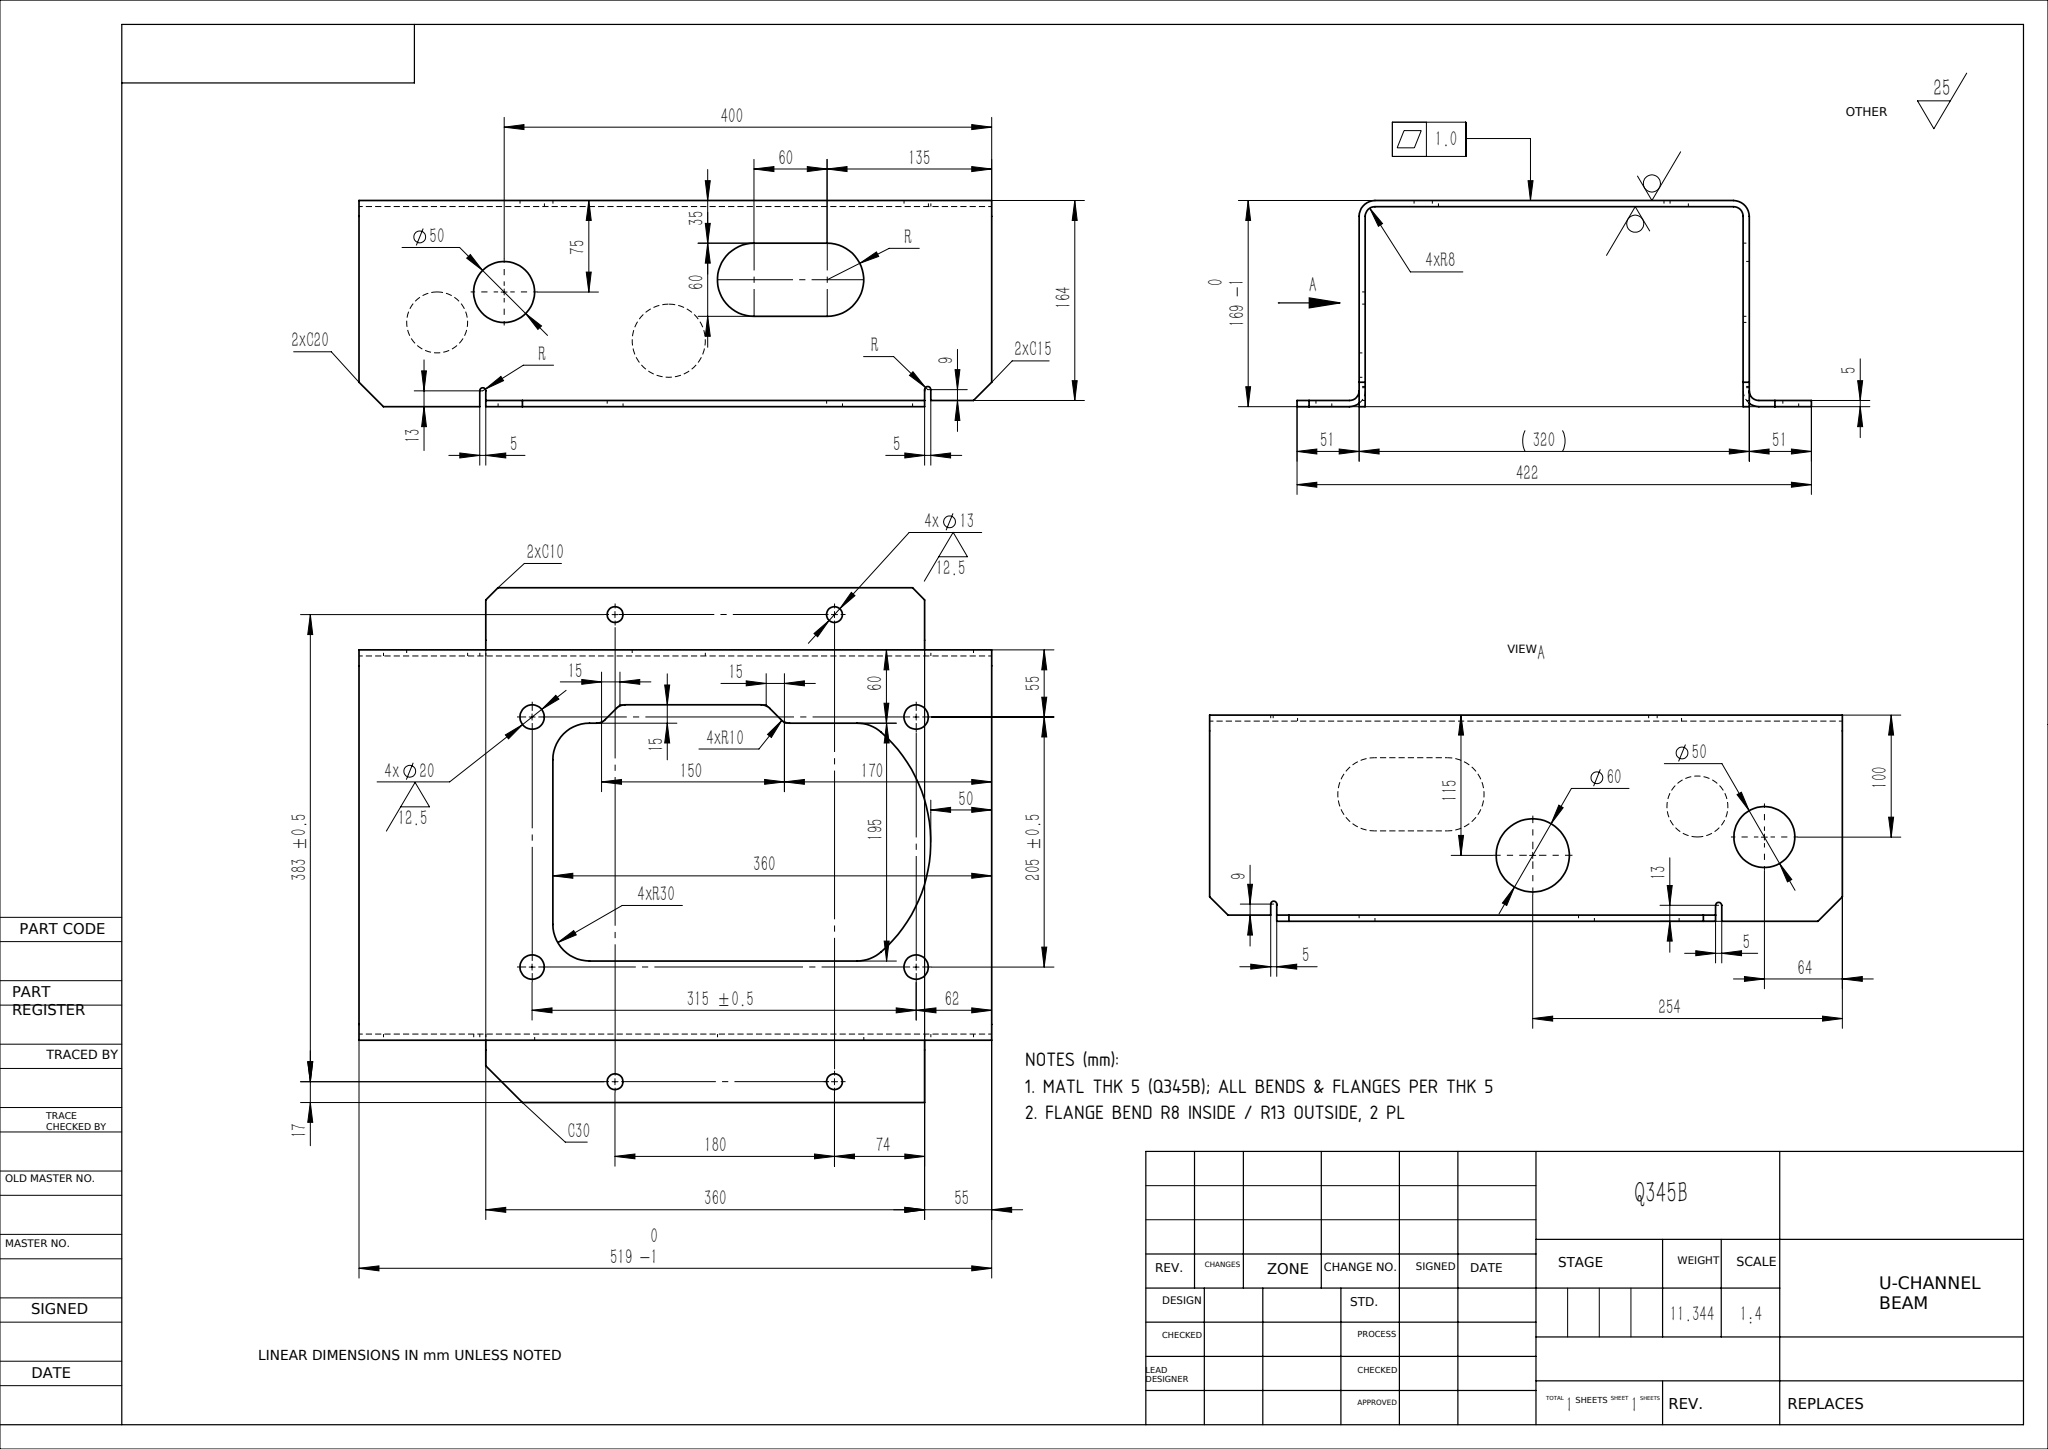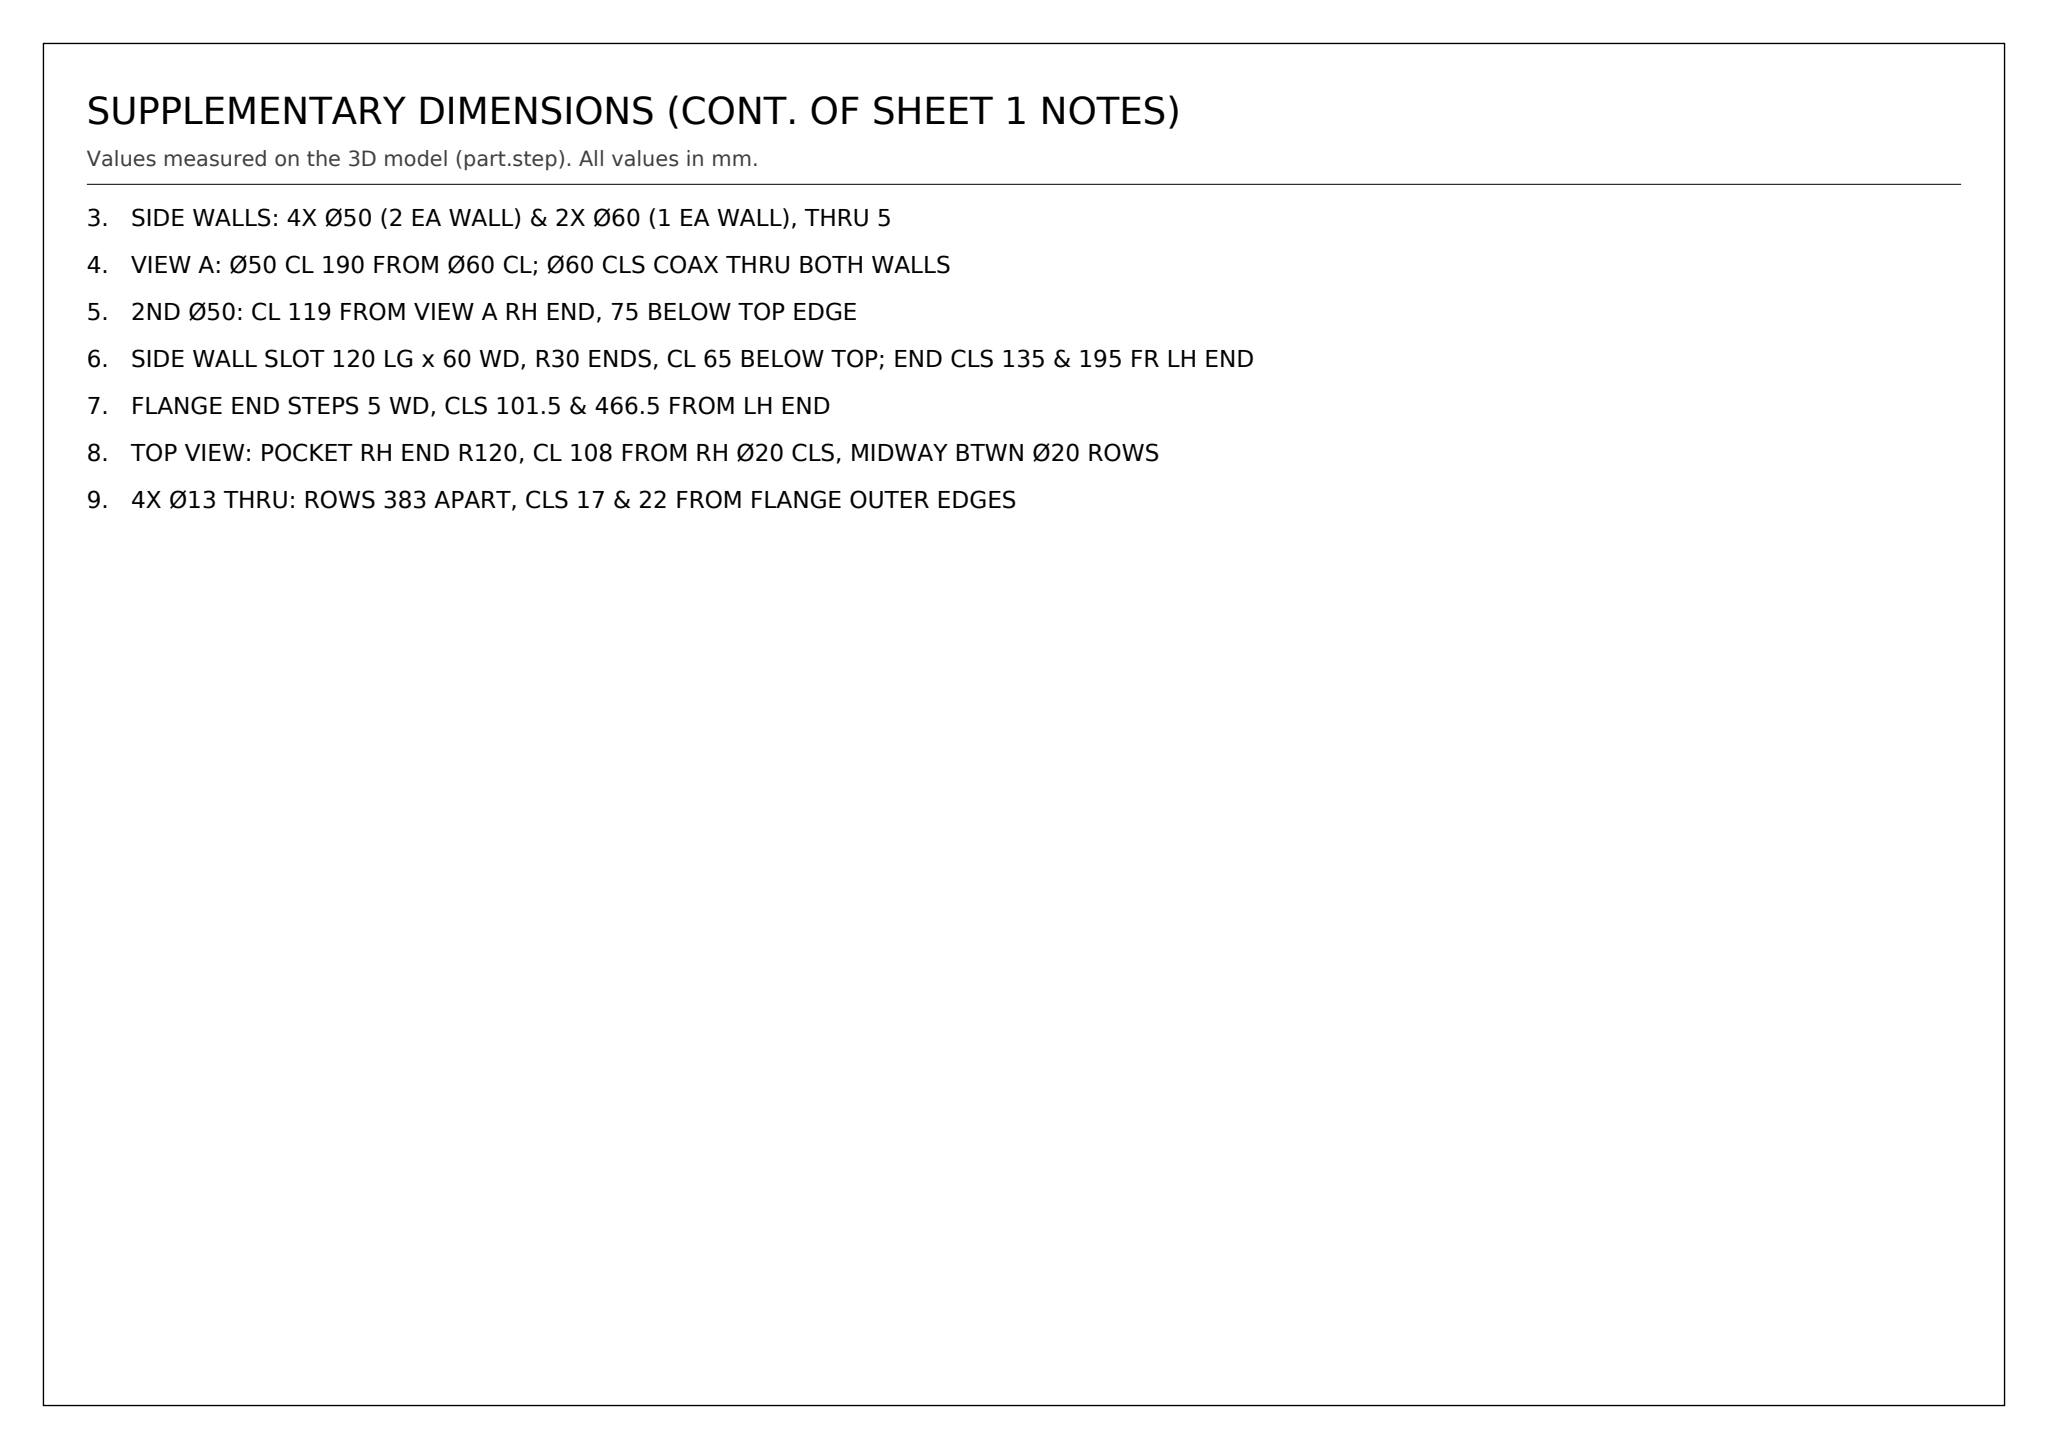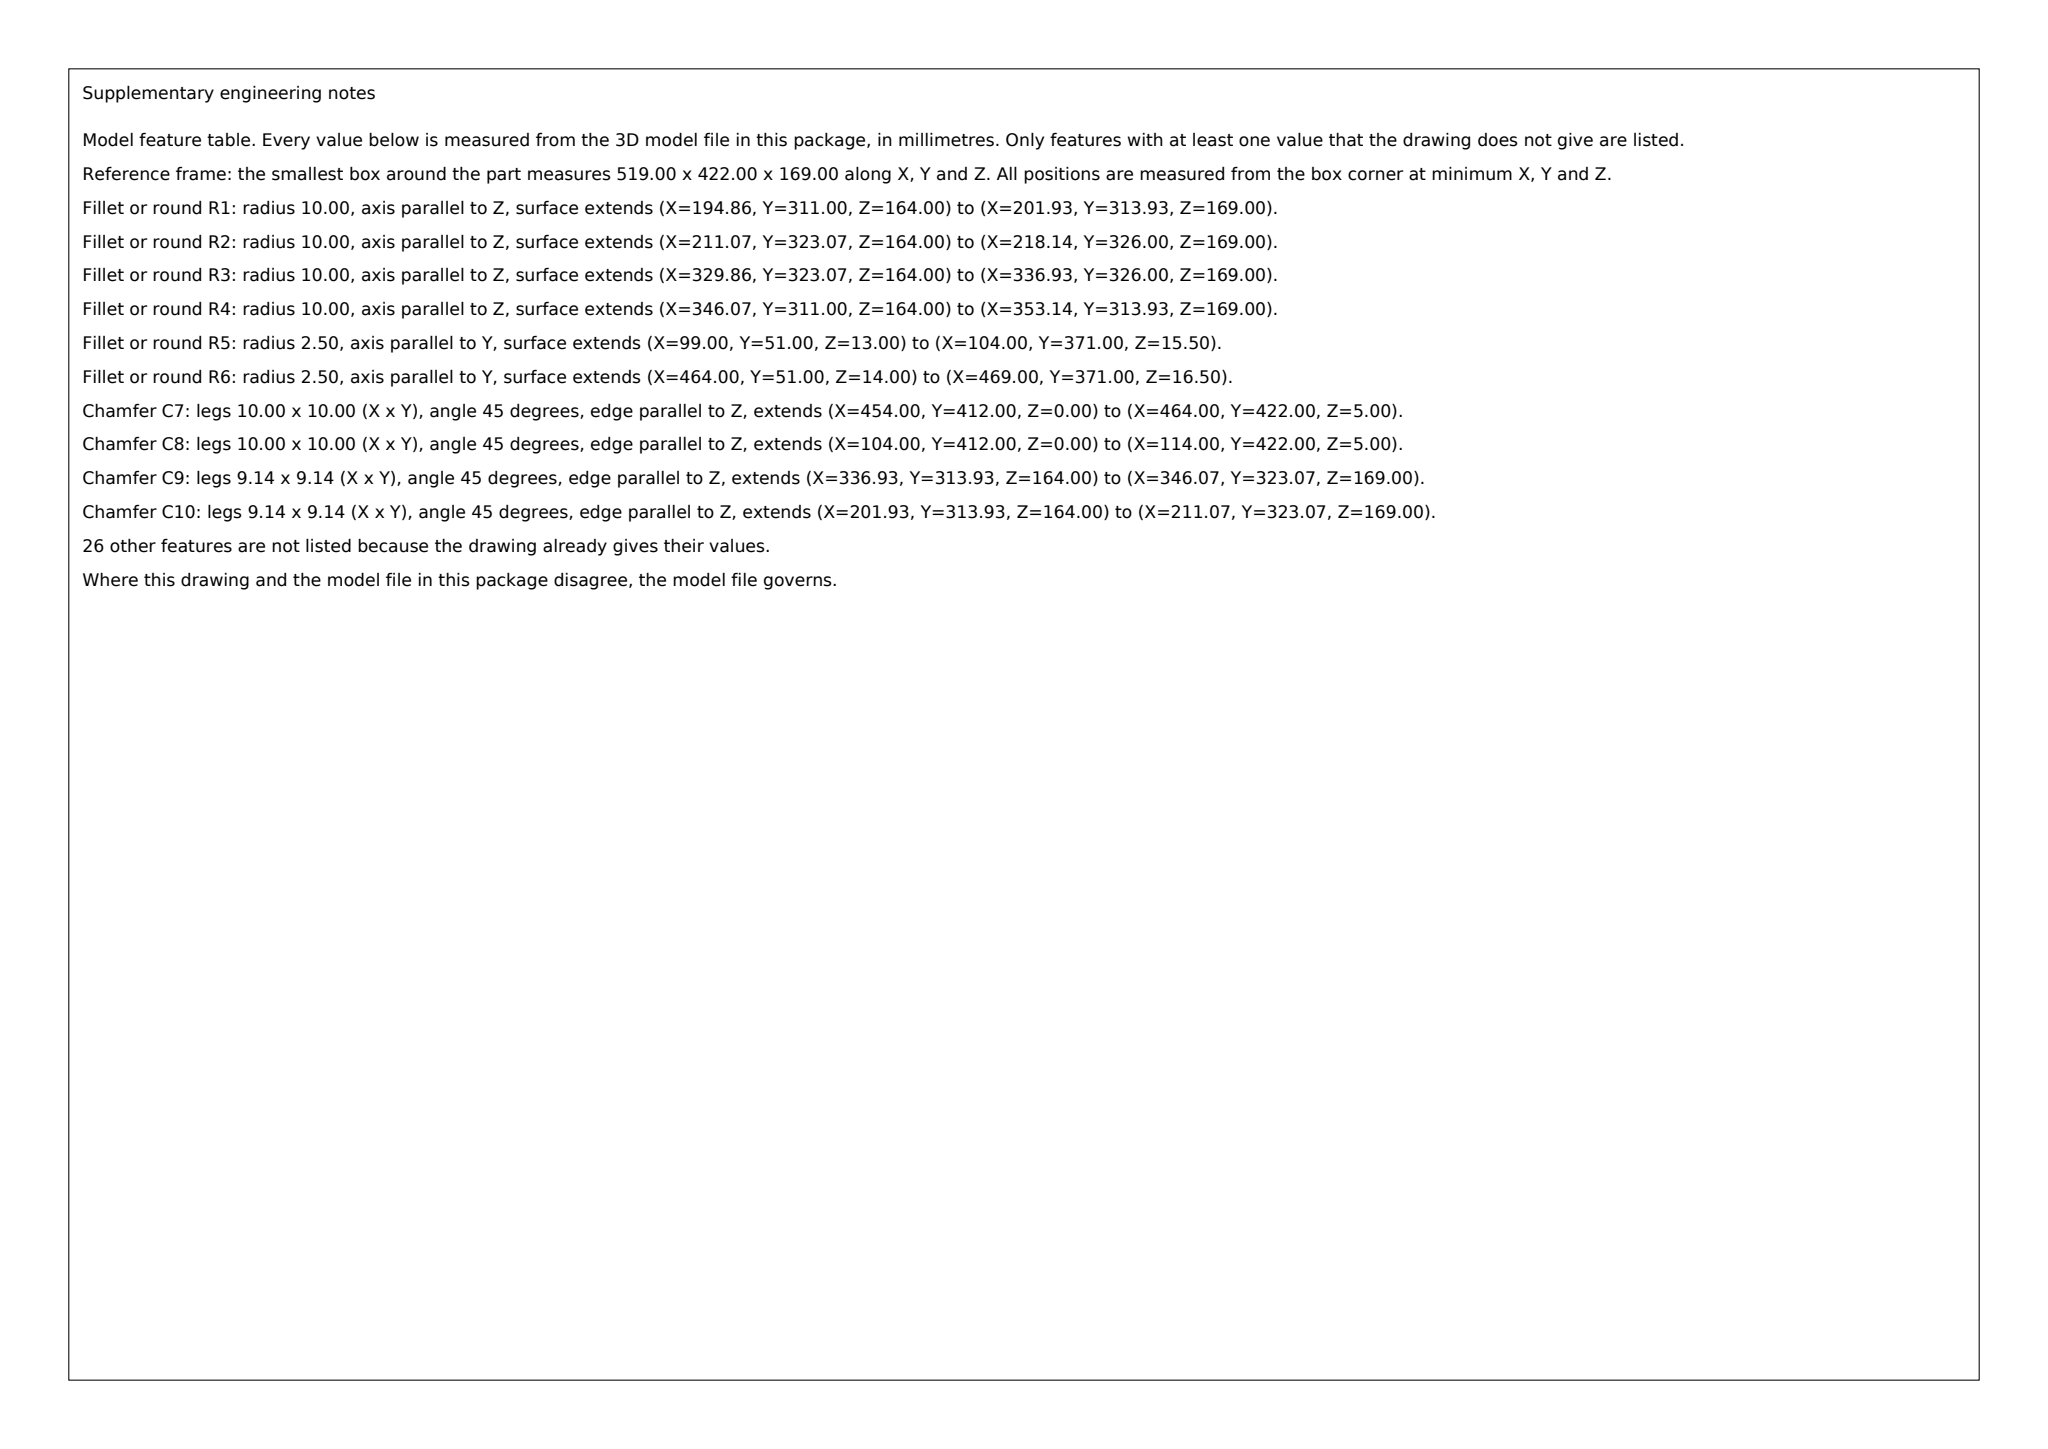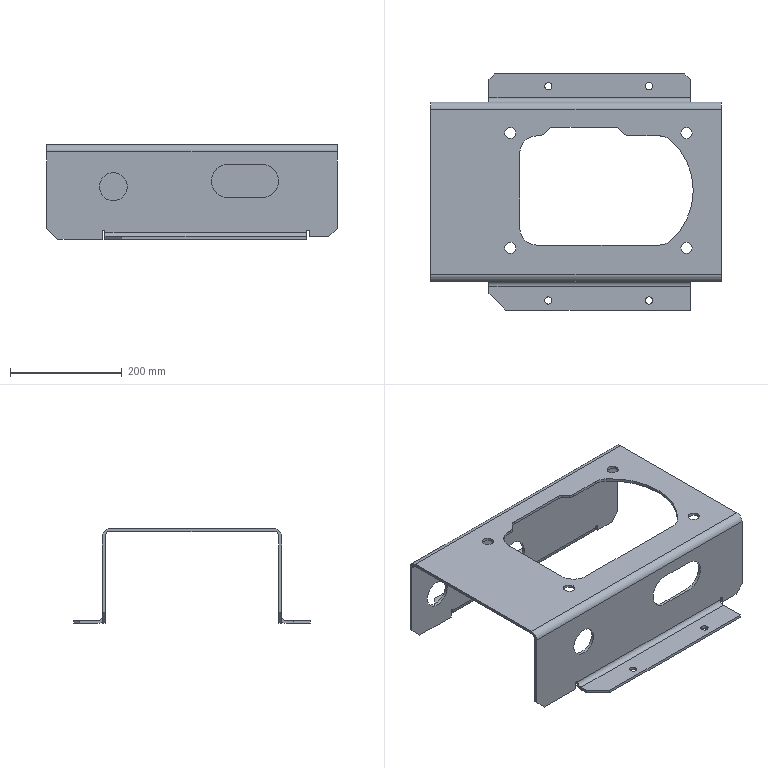Part | SolidWorks | mm | 1 solid | 89 faces | box 519 x 422 x 169 mm | volume 1445072 mm3 | cylinder 47 | plane 42 | commonest cylinder face diameters 20 x12 13 x8 60 x8 5 x6 50 x4 16 x4 26 x4 240 x1
Drawing notes:
MATL THK 5 (Q345B); ALL BENDS & FLANGES PER THK 5 | from the solid: Z planes 0/5 and 164/169 give 5 wall; all hole cyl length = 5.0
FLANGE BEND R8 INSIDE / R13 OUTSIDE, 2 PL | from the solid: x-axis cyls Ø16 & Ø26 at y=43/379, z=13 (bend CLs) -> R8/R13
SIDE WALLS: 4X Ø50 (2 EA WALL) & 2X Ø60 (1 EA WALL), THRU 5 | from the solid: [50,y,[64,-,69],5,count 2], [50,y,[119,-,94],5,count 2], [60,y,[254,-,54],5,count 2]; wall thk 5 (y planes 51/56 and 366/371)
VIEW A: Ø50 CL 190 FROM Ø60 CL; Ø60 CLS COAX THRU BOTH WALLS | from the solid: Ø50 y-axis at x=64, Ø60 y-axis at x=254 -> 190; [60,y,[254,-,54],5,count 2] coaxial pair
2ND Ø50: CL 119 FROM VIEW A RH END, 75 BELOW TOP EDGE | from the solid: Ø50 y-axis cyl pair at x=119, z=94; top edge z=169 -> 169-94=75
SIDE WALL SLOT 120 LG x 60 WD, R30 ENDS, CL 65 BELOW TOP; END CLS 135 & 195 FR LH END | from the solid: Slot end cyls Ø60 axis y at x=324 & x=384 -> R30, 120 overall; CL z=104 (169-104=65); 519-384=135, 519-324=195
FLANGE END STEPS 5 WD, CLS 101.5 & 466.5 FROM LH END | from the solid: x-planes 99/104 and 464/469 (5 wd); Ø5 y-axis features at x=101.5 z=13 and x=466.5 z=14
TOP VIEW: POCKET RH END R120, CL 108 FROM RH Ø20 CLS, MIDWAY BTWN Ø20 ROWS | from the solid: Ø240 z-axis pocket end at x=349, y=213.5 -> R120; RH Ø20 at x=457 -> 108; rows y=111 & 316 midpoint 213.5
4X Ø13 THRU: ROWS 383 APART, CLS 17 & 22 FROM FLANGE OUTER EDGES | from the solid: Ø13 z-axis holes at y=17 and y=400; bbox y=0..422 -> 17 and 22 from edges, 383 apart (x=210 & 390)
build123d program:
from build123d import *

# Parameters (mm, degrees)
SKETCH1_W           = 519
SKETCH1_H           = 320
SKETCH1_R           = 10
BOSS_EXTRUDE1_DEPTH = 5
SKETCH2_W           = 519
SKETCH2_H           = 5
BOSS_EXTRUDE2_DEPTH = 169
SKETCH3_OUTSIDE_W   = 647.542
SKETCH3_OUTSIDE_H   = 297.542
SKETCH3_OUTSIDE_R   = 25
CUT_EXTRUDE4_DEPTH  = 5
SKETCH4_OUTSIDE_W   = 647.542
SKETCH4_OUTSIDE_H   = 297.542
SKETCH4_OUTSIDE_R   = 30
SKETCH4_OUTSIDE_R_2 = 25
CUT_EXTRUDE6_DEPTH  = 5
SKETCH6_W           = 360
SKETCH6_H           = 5
BOSS_EXTRUDE3_DEPTH = 51
SKETCH7_W           = 360
SKETCH7_H           = 5
BOSS_EXTRUDE4_DEPTH = 51
SKETCH8_OUTSIDE_W   = 658.986
SKETCH8_OUTSIDE_H   = 561.986
SKETCH8_OUTSIDE_R   = 6.5
CUT_EXTRUDE8_DEPTH  = 5
FILLET1_R           = 8
FILLET2_R           = 13


with BuildPart() as part:
    # Sketch1 → Boss-Extrude1 (new body)
    with BuildSketch(Plane.XY):
        with Locations((259.5, 160)):
            Rectangle(SKETCH1_W, SKETCH1_H)
        with Locations((142, 265)):
            Circle(SKETCH1_R, mode=Mode.SUBTRACT)
        with Locations((457, 265)):
            Circle(SKETCH1_R, mode=Mode.SUBTRACT)
        with Locations((457, 60)):
            Circle(SKETCH1_R, mode=Mode.SUBTRACT)
        with Locations((142, 60)):
            Circle(SKETCH1_R, mode=Mode.SUBTRACT)
        with BuildLine():
            Line((159, 230), (159, 95))
            ThreePointArc((159, 95), (167.787, 73.787), (189, 65))
            Line((189, 65), (408.529, 65))
            ThreePointArc((408.529, 65), (419.136, 66.938), (428.373, 72.5))
            ThreePointArc((428.373, 72.5), (469, 162.5), (428.373, 252.5))
            ThreePointArc((428.373, 252.5), (419.136, 258.062), (408.529, 260))
            Line((408.529, 260), (353.142, 260))
            ThreePointArc((353.142, 260), (349.315, 260.761), (346.071, 262.929))
            Line((346.071, 262.929), (336.929, 272.071))
            ThreePointArc((336.929, 272.071), (333.685, 274.239), (329.858, 275))
            Line((329.858, 275), (218.142, 275))
            ThreePointArc((218.142, 275), (214.315, 274.239), (211.071, 272.071))
            Line((211.071, 272.071), (201.929, 262.929))
            ThreePointArc((201.929, 262.929), (198.685, 260.761), (194.858, 260))
            Line((194.858, 260), (189, 260))
            ThreePointArc((189, 260), (167.787, 251.213), (159, 230))
        make_face(mode=Mode.SUBTRACT)
    extrude(amount=BOSS_EXTRUDE1_DEPTH)

    # Sketch2 → Boss-Extrude2 (add)
    with BuildSketch(Plane.XY.offset(5)):
        with Locations((259.5, 317.5)):
            Rectangle(SKETCH2_W, SKETCH2_H)
        with Locations((259.5, 2.5)):
            Rectangle(SKETCH2_W, SKETCH2_H)
    extrude(amount=-BOSS_EXTRUDE2_DEPTH)

    # Sketch3 outside → Cut-Extrude4 (cut)
    # profile 1 of 3: a face of its own
    with BuildSketch(Plane(origin=(0, 0, 0), x_dir=(-1, 0, 0), z_dir=(0, -1, 0))):
        with Locations((-259.5, 79.5)):
            Rectangle(SKETCH3_OUTSIDE_W, SKETCH3_OUTSIDE_H)
        with BuildLine():
            Line((0, 144), (-20, 164))
            Line((-20, 164), (-99, 164))
            Line((-99, 164), (-99, 151))
            ThreePointArc((-99, 151), (-101.5, 148.5), (-104, 151))
            Line((-104, 151), (-104, 164))
            Line((-104, 164), (-464, 164))
            Line((-464, 164), (-464, 150))
            ThreePointArc((-464, 150), (-466.5, 147.5), (-469, 150))
            Line((-469, 150), (-469, 164))
            Line((-469, 164), (-499, 164))
            Line((-499, 164), (-519, 144))
            Line((-519, 144), (-519, -5))
            Line((-519, -5), (0, -5))
            Line((0, -5), (0, 144))
        make_face(mode=Mode.SUBTRACT)
    # profile 2 of 3: a face of its own
    with BuildSketch(Plane(origin=(0, 0, 0), x_dir=(-1, 0, 0), z_dir=(0, -1, 0))):
        with Locations(Location((-119, 70, 0), (0, 0, 90))):
            Circle(SKETCH3_OUTSIDE_R)
    # profile 3 of 3: a face of its own
    with BuildSketch(Plane(origin=(0, 0, 0), x_dir=(-1, 0, 0), z_dir=(0, -1, 0))):
        with BuildLine():
            Line((-324, 30), (-384, 30))
            ThreePointArc((-384, 30), (-414, 60), (-384, 90))
            Line((-384, 90), (-324, 90))
            ThreePointArc((-324, 90), (-294, 60), (-324, 30))
        make_face()
    extrude(amount=-CUT_EXTRUDE4_DEPTH, mode=Mode.SUBTRACT)

    # Sketch4 outside → Cut-Extrude6 (cut)
    # profile 1 of 3: a face of its own
    with BuildSketch(Plane(origin=(0, 320, 0), x_dir=(1, 0, 0), z_dir=(0, 1, 0))):
        with Locations((259.5, 79.5)):
            Rectangle(SKETCH4_OUTSIDE_W, SKETCH4_OUTSIDE_H)
        with BuildLine():
            Line((469, 164), (469, 150))
            ThreePointArc((469, 150), (466.5, 147.5), (464, 150))
            Line((464, 150), (464, 164))
            Line((464, 164), (104, 164))
            Line((104, 164), (104, 151))
            ThreePointArc((104, 151), (101.5, 148.5), (99, 151))
            Line((99, 151), (99, 164))
            Line((99, 164), (20, 164))
            Line((20, 164), (0, 144))
            Line((0, 144), (0, -5))
            Line((0, -5), (519, -5))
            Line((519, -5), (519, 144))
            Line((519, 144), (499, 164))
            Line((499, 164), (469, 164))
        make_face(mode=Mode.SUBTRACT)
    # profile 2 of 3: a face of its own
    with BuildSketch(Plane(origin=(0, 320, 0), x_dir=(1, 0, 0), z_dir=(0, 1, 0))):
        with Locations(Location((254, 110, 0), (0, 0, 270))):
            Circle(SKETCH4_OUTSIDE_R)
    # profile 3 of 3: a face of its own
    with BuildSketch(Plane(origin=(0, 320, 0), x_dir=(1, 0, 0), z_dir=(0, 1, 0))):
        with Locations(Location((64, 95, 0), (0, 0, 270))):
            Circle(SKETCH4_OUTSIDE_R_2)
    extrude(amount=-CUT_EXTRUDE6_DEPTH, mode=Mode.SUBTRACT)

    # Sketch6 → Boss-Extrude3 (add)
    with BuildSketch(Plane(origin=(0, 0, 0), x_dir=(-1, 0, 0), z_dir=(0, -1, 0))):
        with Locations((-284, 161.5)):
            Rectangle(SKETCH6_W, SKETCH6_H)
    extrude(amount=BOSS_EXTRUDE3_DEPTH)

    # Sketch7 → Boss-Extrude4 (add)
    with BuildSketch(Plane(origin=(0, 320, 0), x_dir=(1, 0, 0), z_dir=(0, 1, 0))):
        with Locations((284, 161.5)):
            Rectangle(SKETCH7_W, SKETCH7_H)
    extrude(amount=BOSS_EXTRUDE4_DEPTH)

    # Sketch8 outside → Cut-Extrude8 (cut)
    # profile 1 of 5: a face of its own
    with BuildSketch(Plane.XY.offset(-159)):
        with Locations((259.5, 160)):
            Rectangle(SKETCH8_OUTSIDE_W, SKETCH8_OUTSIDE_H)
        Polygon((104, 361), (114, 371), (454, 371), (464, 361), (464, 315), (0, 315), (0, 320), (104, 320), align=None, mode=Mode.SUBTRACT)
        Polygon((134, -51), (464, -51), (464, 5), (0, 5), (0, 0), (104, 0), (104, -21), align=None, mode=Mode.SUBTRACT)
    # profile 2 of 5: a face of its own
    with BuildSketch(Plane.XY.offset(-159)):
        with Locations((210, 349)):
            Circle(SKETCH8_OUTSIDE_R)
    # profile 3 of 5: a face of its own
    with BuildSketch(Plane.XY.offset(-159)):
        with Locations((390, 349)):
            Circle(SKETCH8_OUTSIDE_R)
    # profile 4 of 5: a face of its own
    with BuildSketch(Plane.XY.offset(-159)):
        with Locations((210, -34)):
            Circle(SKETCH8_OUTSIDE_R)
    # profile 5 of 5: a face of its own
    with BuildSketch(Plane.XY.offset(-159)):
        with Locations((390, -34)):
            Circle(SKETCH8_OUTSIDE_R)
    extrude(amount=-CUT_EXTRUDE8_DEPTH, mode=Mode.SUBTRACT)

    # Fillet1
    fillet1_edges = [part.edges().sort_by_distance(p)[0] for p in [
        (284, 320, -159),
        (284, 0, -159),
        (259.5, 5, 0),
        (259.5, 315, 0),
    ]]
    fillet(fillet1_edges, radius=FILLET1_R)

    # Fillet2
    fillet2_edges = [part.edges().sort_by_distance(p)[0] for p in [
        (259.5, 320, 5),
        (284, 5, -164),
        (284, 315, -164),
        (259.5, 0, 5),
    ]]
    fillet(fillet2_edges, radius=FILLET2_R)


solid = part.part